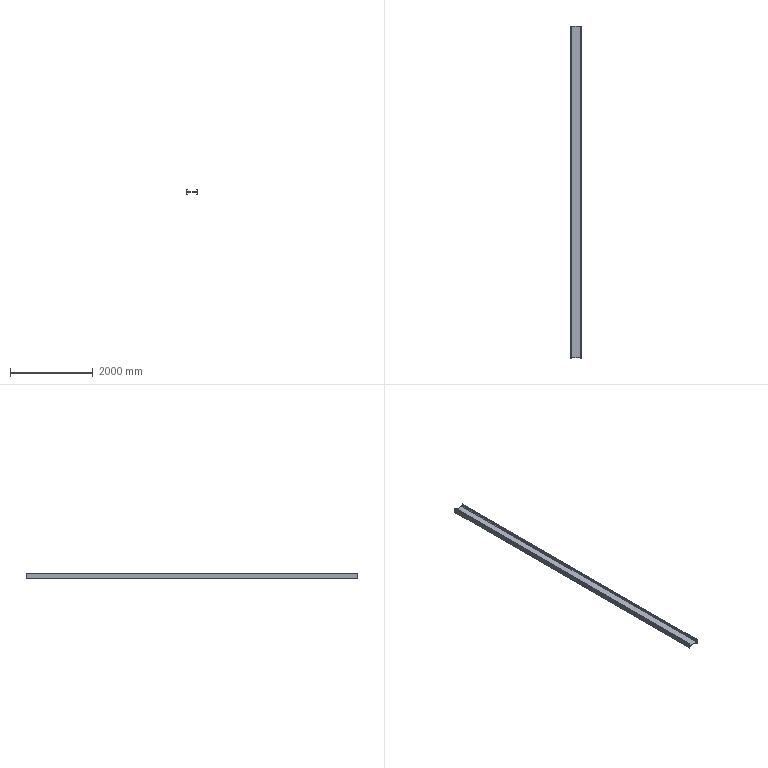Component | SolidWorks | H250X125-7375-16 | 1 solid | 18 faces | box 250 x 8000 x 125 mm | volume 30296567 mm3 | plane 14 | cylinder 4 | commonest cylinder face diameters 26 x4
build123d program:
from build123d import *

# Parameters (mm, degrees)
H_BEAM_HN250_125_1_DEPTH = 8000


with BuildPart() as part:
    # Sketch1 → H-Beam HN250_125_1 (new body)
    with BuildSketch(Plane.YZ):
        with BuildLine():
            Line((-62.5, -125), (-62.5, -116))
            Line((-62.5, -116), (-16, -116))
            ThreePointArc((-16, -116), (-6.808, -112.192), (-3, -103))
            Line((-3, -103), (-3, 103))
            ThreePointArc((-3, 103), (-6.808, 112.192), (-16, 116))
            Line((-16, 116), (-62.5, 116))
            Line((-62.5, 116), (-62.5, 125))
            Line((-62.5, 125), (62.5, 125))
            Line((62.5, 125), (62.5, 116))
            Line((62.5, 116), (16, 116))
            ThreePointArc((16, 116), (6.808, 112.192), (3, 103))
            Line((3, 103), (3, -103))
            ThreePointArc((3, -103), (6.808, -112.192), (16, -116))
            Line((16, -116), (62.5, -116))
            Line((62.5, -116), (62.5, -125))
            Line((62.5, -125), (-62.5, -125))
        make_face()
    extrude(amount=H_BEAM_HN250_125_1_DEPTH)


solid = part.part

# Placed as in the assembly
solid = solid.moved(Location((1944.926, 805.154, 161.5), (90, -90, 0)))
STEP:
#1=COLOUR_RGB('',0.7922,0.8196,0.9333);
#2=FILL_AREA_STYLE_COLOUR('',#1);
#3=FILL_AREA_STYLE('',(#2));
#4=SURFACE_STYLE_FILL_AREA(#3);
#5=SURFACE_SIDE_STYLE('',(#4));
#6=SURFACE_STYLE_USAGE(.BOTH.,#5);
#7=PRESENTATION_STYLE_ASSIGNMENT((#6));
#8=CARTESIAN_POINT('',(71.651,-283.262,3.898));
#9=VERTEX_POINT('',#8);
#10=CARTESIAN_POINT('',(71.651,-283.262,8.819));
#11=VERTEX_POINT('',#10);
#12=CARTESIAN_POINT('',(71.651,-283.262,8.819));
#13=DIRECTION('',(0.,0.,1.));
#14=VECTOR('',#13,39.37);
#15=LINE('',#12,#14);
#16=EDGE_CURVE('',#9,#11,#15,.T.);
#17=ORIENTED_EDGE('',*,*,#16,.T.);
#18=CARTESIAN_POINT('',(71.651,31.699,8.819));
#19=VERTEX_POINT('',#18);
#20=CARTESIAN_POINT('',(71.651,31.699,8.819));
#21=DIRECTION('',(-0.,-1.,0.));
#22=VECTOR('',#21,39.37);
#23=LINE('',#20,#22);
#24=EDGE_CURVE('',#19,#11,#23,.T.);
#25=ORIENTED_EDGE('',*,*,#24,.F.);
#26=CARTESIAN_POINT('',(71.651,31.699,3.898));
#27=VERTEX_POINT('',#26);
#28=CARTESIAN_POINT('',(71.651,31.699,8.819));
#29=DIRECTION('',(0.,0.,1.));
#30=VECTOR('',#29,39.37);
#31=LINE('',#28,#30);
#32=EDGE_CURVE('',#27,#19,#31,.T.);
#33=ORIENTED_EDGE('',*,*,#32,.F.);
#34=CARTESIAN_POINT('',(71.651,31.699,3.898));
#35=DIRECTION('',(-0.,-1.,0.));
#36=VECTOR('',#35,39.37);
#37=LINE('',#34,#36);
#38=EDGE_CURVE('',#27,#9,#37,.T.);
#39=ORIENTED_EDGE('',*,*,#38,.T.);
#40=EDGE_LOOP('',(#17,#25,#33,#39));
#41=FACE_OUTER_BOUND('',#40,.T.);
#42=CARTESIAN_POINT('',(71.651,31.699,8.819));
#43=DIRECTION('',(1.,-0.,-0.));
#44=DIRECTION('',(0.,1.,-0.));
#45=AXIS2_PLACEMENT_3D('',#42,#43,#44);
#46=PLANE('',#45);
#47=ADVANCED_FACE('',(#41),#46,.F.);
#48=CARTESIAN_POINT('',(72.005,-283.262,8.819));
#49=VERTEX_POINT('',#48);
#50=CARTESIAN_POINT('',(72.005,-283.262,8.819));
#51=DIRECTION('',(1.,-0.,-0.));
#52=VECTOR('',#51,39.37);
#53=LINE('',#50,#52);
#54=EDGE_CURVE('',#11,#49,#53,.T.);
#55=ORIENTED_EDGE('',*,*,#54,.T.);
#56=CARTESIAN_POINT('',(72.005,31.699,8.819));
#57=VERTEX_POINT('',#56);
#58=CARTESIAN_POINT('',(72.005,31.699,8.819));
#59=DIRECTION('',(-0.,-1.,0.));
#60=VECTOR('',#59,39.37);
#61=LINE('',#58,#60);
#62=EDGE_CURVE('',#57,#49,#61,.T.);
#63=ORIENTED_EDGE('',*,*,#62,.F.);
#64=CARTESIAN_POINT('',(72.005,31.699,8.819));
#65=DIRECTION('',(1.,-0.,-0.));
#66=VECTOR('',#65,39.37);
#67=LINE('',#64,#66);
#68=EDGE_CURVE('',#19,#57,#67,.T.);
#69=ORIENTED_EDGE('',*,*,#68,.F.);
#70=ORIENTED_EDGE('',*,*,#24,.T.);
#71=EDGE_LOOP('',(#55,#63,#69,#70));
#72=FACE_OUTER_BOUND('',#71,.T.);
#73=CARTESIAN_POINT('',(72.005,31.699,8.819));
#74=DIRECTION('',(-0.,-0.,-1.));
#75=DIRECTION('',(-1.,0.,0.));
#76=AXIS2_PLACEMENT_3D('',#73,#74,#75);
#77=PLANE('',#76);
#78=ADVANCED_FACE('',(#72),#77,.F.);
#79=CARTESIAN_POINT('',(72.005,-283.262,6.988));
#80=VERTEX_POINT('',#79);
#81=CARTESIAN_POINT('',(72.005,-283.262,8.819));
#82=DIRECTION('',(0.,-0.,-1.));
#83=VECTOR('',#82,39.37);
#84=LINE('',#81,#83);
#85=EDGE_CURVE('',#49,#80,#84,.T.);
#86=ORIENTED_EDGE('',*,*,#85,.T.);
#87=CARTESIAN_POINT('',(72.005,31.699,6.988));
#88=VERTEX_POINT('',#87);
#89=CARTESIAN_POINT('',(72.005,31.699,6.988));
#90=DIRECTION('',(-0.,-1.,0.));
#91=VECTOR('',#90,39.37);
#92=LINE('',#89,#91);
#93=EDGE_CURVE('',#88,#80,#92,.T.);
#94=ORIENTED_EDGE('',*,*,#93,.F.);
#95=CARTESIAN_POINT('',(72.005,31.699,8.819));
#96=DIRECTION('',(0.,-0.,-1.));
#97=VECTOR('',#96,39.37);
#98=LINE('',#95,#97);
#99=EDGE_CURVE('',#57,#88,#98,.T.);
#100=ORIENTED_EDGE('',*,*,#99,.F.);
#101=ORIENTED_EDGE('',*,*,#62,.T.);
#102=EDGE_LOOP('',(#86,#94,#100,#101));
#103=FACE_OUTER_BOUND('',#102,.T.);
#104=CARTESIAN_POINT('',(72.005,31.699,8.819));
#105=DIRECTION('',(-1.,0.,-0.));
#106=DIRECTION('',(-0.,0.,1.));
#107=AXIS2_PLACEMENT_3D('',#104,#105,#106);
#108=PLANE('',#107);
#109=ADVANCED_FACE('',(#103),#108,.F.);
#110=CARTESIAN_POINT('',(72.517,-283.262,6.476));
#111=VERTEX_POINT('',#110);
#112=CARTESIAN_POINT('',(72.517,-283.262,6.988));
#113=DIRECTION('',(-0.,-1.,0.));
#114=DIRECTION('',(1.,0.,0.));
#115=AXIS2_PLACEMENT_3D('',#112,#113,#114);
#116=CIRCLE('',#115,0.5118);
#117=EDGE_CURVE('',#80,#111,#116,.T.);
#118=ORIENTED_EDGE('',*,*,#117,.T.);
#119=CARTESIAN_POINT('',(72.517,31.699,6.476));
#120=VERTEX_POINT('',#119);
#121=CARTESIAN_POINT('',(72.517,31.699,6.476));
#122=DIRECTION('',(-0.,-1.,0.));
#123=VECTOR('',#122,39.37);
#124=LINE('',#121,#123);
#125=EDGE_CURVE('',#120,#111,#124,.T.);
#126=ORIENTED_EDGE('',*,*,#125,.F.);
#127=CARTESIAN_POINT('',(72.517,31.699,6.988));
#128=DIRECTION('',(-0.,-1.,0.));
#129=DIRECTION('',(1.,0.,0.));
#130=AXIS2_PLACEMENT_3D('',#127,#128,#129);
#131=CIRCLE('',#130,0.5118);
#132=EDGE_CURVE('',#88,#120,#131,.T.);
#133=ORIENTED_EDGE('',*,*,#132,.F.);
#134=ORIENTED_EDGE('',*,*,#93,.T.);
#135=EDGE_LOOP('',(#118,#126,#133,#134));
#136=FACE_OUTER_BOUND('',#135,.T.);
#137=CARTESIAN_POINT('',(72.517,31.699,6.988));
#138=DIRECTION('',(-0.,-1.,0.));
#139=DIRECTION('',(1.,0.,0.));
#140=AXIS2_PLACEMENT_3D('',#137,#138,#139);
#141=CYLINDRICAL_SURFACE('',#140,0.5118);
#142=ADVANCED_FACE('',(#136),#141,.F.);
#143=CARTESIAN_POINT('',(80.627,-283.262,6.476));
#144=VERTEX_POINT('',#143);
#145=CARTESIAN_POINT('',(80.627,-283.262,6.476));
#146=DIRECTION('',(1.,-0.,-0.));
#147=VECTOR('',#146,39.37);
#148=LINE('',#145,#147);
#149=EDGE_CURVE('',#111,#144,#148,.T.);
#150=ORIENTED_EDGE('',*,*,#149,.T.);
#151=CARTESIAN_POINT('',(80.627,31.699,6.476));
#152=VERTEX_POINT('',#151);
#153=CARTESIAN_POINT('',(80.627,31.699,6.476));
#154=DIRECTION('',(-0.,-1.,0.));
#155=VECTOR('',#154,39.37);
#156=LINE('',#153,#155);
#157=EDGE_CURVE('',#152,#144,#156,.T.);
#158=ORIENTED_EDGE('',*,*,#157,.F.);
#159=CARTESIAN_POINT('',(80.627,31.699,6.476));
#160=DIRECTION('',(1.,-0.,-0.));
#161=VECTOR('',#160,39.37);
#162=LINE('',#159,#161);
#163=EDGE_CURVE('',#120,#152,#162,.T.);
#164=ORIENTED_EDGE('',*,*,#163,.F.);
#165=ORIENTED_EDGE('',*,*,#125,.T.);
#166=EDGE_LOOP('',(#150,#158,#164,#165));
#167=FACE_OUTER_BOUND('',#166,.T.);
#168=CARTESIAN_POINT('',(80.627,31.699,6.476));
#169=DIRECTION('',(-0.,-0.,-1.));
#170=DIRECTION('',(-1.,0.,0.));
#171=AXIS2_PLACEMENT_3D('',#168,#169,#170);
#172=PLANE('',#171);
#173=ADVANCED_FACE('',(#167),#172,.F.);
#174=CARTESIAN_POINT('',(81.139,-283.262,6.988));
#175=VERTEX_POINT('',#174);
#176=CARTESIAN_POINT('',(80.627,-283.262,6.988));
#177=DIRECTION('',(-0.,-1.,0.));
#178=DIRECTION('',(1.,0.,0.));
#179=AXIS2_PLACEMENT_3D('',#176,#177,#178);
#180=CIRCLE('',#179,0.5118);
#181=EDGE_CURVE('',#144,#175,#180,.T.);
#182=ORIENTED_EDGE('',*,*,#181,.T.);
#183=CARTESIAN_POINT('',(81.139,31.699,6.988));
#184=VERTEX_POINT('',#183);
#185=CARTESIAN_POINT('',(81.139,31.699,6.988));
#186=DIRECTION('',(-0.,-1.,0.));
#187=VECTOR('',#186,39.37);
#188=LINE('',#185,#187);
#189=EDGE_CURVE('',#184,#175,#188,.T.);
#190=ORIENTED_EDGE('',*,*,#189,.F.);
#191=CARTESIAN_POINT('',(80.627,31.699,6.988));
#192=DIRECTION('',(-0.,-1.,0.));
#193=DIRECTION('',(1.,0.,0.));
#194=AXIS2_PLACEMENT_3D('',#191,#192,#193);
#195=CIRCLE('',#194,0.5118);
#196=EDGE_CURVE('',#152,#184,#195,.T.);
#197=ORIENTED_EDGE('',*,*,#196,.F.);
#198=ORIENTED_EDGE('',*,*,#157,.T.);
#199=EDGE_LOOP('',(#182,#190,#197,#198));
#200=FACE_OUTER_BOUND('',#199,.T.);
#201=CARTESIAN_POINT('',(80.627,31.699,6.988));
#202=DIRECTION('',(-0.,-1.,0.));
#203=DIRECTION('',(1.,0.,0.));
#204=AXIS2_PLACEMENT_3D('',#201,#202,#203);
#205=CYLINDRICAL_SURFACE('',#204,0.5118);
#206=ADVANCED_FACE('',(#200),#205,.F.);
#207=CARTESIAN_POINT('',(81.139,-283.262,8.819));
#208=VERTEX_POINT('',#207);
#209=CARTESIAN_POINT('',(81.139,-283.262,6.988));
#210=DIRECTION('',(0.,0.,1.));
#211=VECTOR('',#210,39.37);
#212=LINE('',#209,#211);
#213=EDGE_CURVE('',#175,#208,#212,.T.);
#214=ORIENTED_EDGE('',*,*,#213,.T.);
#215=CARTESIAN_POINT('',(81.139,31.699,8.819));
#216=VERTEX_POINT('',#215);
#217=CARTESIAN_POINT('',(81.139,31.699,8.819));
#218=DIRECTION('',(-0.,-1.,0.));
#219=VECTOR('',#218,39.37);
#220=LINE('',#217,#219);
#221=EDGE_CURVE('',#216,#208,#220,.T.);
#222=ORIENTED_EDGE('',*,*,#221,.F.);
#223=CARTESIAN_POINT('',(81.139,31.699,6.988));
#224=DIRECTION('',(0.,0.,1.));
#225=VECTOR('',#224,39.37);
#226=LINE('',#223,#225);
#227=EDGE_CURVE('',#184,#216,#226,.T.);
#228=ORIENTED_EDGE('',*,*,#227,.F.);
#229=ORIENTED_EDGE('',*,*,#189,.T.);
#230=EDGE_LOOP('',(#214,#222,#228,#229));
#231=FACE_OUTER_BOUND('',#230,.T.);
#232=CARTESIAN_POINT('',(81.139,31.699,6.988));
#233=DIRECTION('',(1.,-0.,-0.));
#234=DIRECTION('',(0.,1.,-0.));
#235=AXIS2_PLACEMENT_3D('',#232,#233,#234);
#236=PLANE('',#235);
#237=ADVANCED_FACE('',(#231),#236,.F.);
#238=CARTESIAN_POINT('',(81.493,-283.262,8.819));
#239=VERTEX_POINT('',#238);
#240=CARTESIAN_POINT('',(81.493,-283.262,8.819));
#241=DIRECTION('',(1.,-0.,-0.));
#242=VECTOR('',#241,39.37);
#243=LINE('',#240,#242);
#244=EDGE_CURVE('',#208,#239,#243,.T.);
#245=ORIENTED_EDGE('',*,*,#244,.T.);
#246=CARTESIAN_POINT('',(81.493,31.699,8.819));
#247=VERTEX_POINT('',#246);
#248=CARTESIAN_POINT('',(81.493,31.699,8.819));
#249=DIRECTION('',(-0.,-1.,0.));
#250=VECTOR('',#249,39.37);
#251=LINE('',#248,#250);
#252=EDGE_CURVE('',#247,#239,#251,.T.);
#253=ORIENTED_EDGE('',*,*,#252,.F.);
#254=CARTESIAN_POINT('',(81.493,31.699,8.819));
#255=DIRECTION('',(1.,-0.,-0.));
#256=VECTOR('',#255,39.37);
#257=LINE('',#254,#256);
#258=EDGE_CURVE('',#216,#247,#257,.T.);
#259=ORIENTED_EDGE('',*,*,#258,.F.);
#260=ORIENTED_EDGE('',*,*,#221,.T.);
#261=EDGE_LOOP('',(#245,#253,#259,#260));
#262=FACE_OUTER_BOUND('',#261,.T.);
#263=CARTESIAN_POINT('',(81.493,31.699,8.819));
#264=DIRECTION('',(-0.,-0.,-1.));
#265=DIRECTION('',(-1.,0.,0.));
#266=AXIS2_PLACEMENT_3D('',#263,#264,#265);
#267=PLANE('',#266);
#268=ADVANCED_FACE('',(#262),#267,.F.);
#269=CARTESIAN_POINT('',(81.493,-283.262,3.898));
#270=VERTEX_POINT('',#269);
#271=CARTESIAN_POINT('',(81.493,-283.262,3.898));
#272=DIRECTION('',(-0.,-0.,-1.));
#273=VECTOR('',#272,39.37);
#274=LINE('',#271,#273);
#275=EDGE_CURVE('',#239,#270,#274,.T.);
#276=ORIENTED_EDGE('',*,*,#275,.T.);
#277=CARTESIAN_POINT('',(81.493,31.699,3.898));
#278=VERTEX_POINT('',#277);
#279=CARTESIAN_POINT('',(81.493,31.699,3.898));
#280=DIRECTION('',(-0.,-1.,0.));
#281=VECTOR('',#280,39.37);
#282=LINE('',#279,#281);
#283=EDGE_CURVE('',#278,#270,#282,.T.);
#284=ORIENTED_EDGE('',*,*,#283,.F.);
#285=CARTESIAN_POINT('',(81.493,31.699,3.898));
#286=DIRECTION('',(-0.,-0.,-1.));
#287=VECTOR('',#286,39.37);
#288=LINE('',#285,#287);
#289=EDGE_CURVE('',#247,#278,#288,.T.);
#290=ORIENTED_EDGE('',*,*,#289,.F.);
#291=ORIENTED_EDGE('',*,*,#252,.T.);
#292=EDGE_LOOP('',(#276,#284,#290,#291));
#293=FACE_OUTER_BOUND('',#292,.T.);
#294=CARTESIAN_POINT('',(81.493,31.699,3.898));
#295=DIRECTION('',(-1.,0.,0.));
#296=DIRECTION('',(-0.,-1.,0.));
#297=AXIS2_PLACEMENT_3D('',#294,#295,#296);
#298=PLANE('',#297);
#299=ADVANCED_FACE('',(#293),#298,.F.);
#300=CARTESIAN_POINT('',(81.139,-283.262,3.898));
#301=VERTEX_POINT('',#300);
#302=CARTESIAN_POINT('',(81.139,-283.262,3.898));
#303=DIRECTION('',(-1.,0.,0.));
#304=VECTOR('',#303,39.37);
#305=LINE('',#302,#304);
#306=EDGE_CURVE('',#270,#301,#305,.T.);
#307=ORIENTED_EDGE('',*,*,#306,.T.);
#308=CARTESIAN_POINT('',(81.139,31.699,3.898));
#309=VERTEX_POINT('',#308);
#310=CARTESIAN_POINT('',(81.139,31.699,3.898));
#311=DIRECTION('',(-0.,-1.,0.));
#312=VECTOR('',#311,39.37);
#313=LINE('',#310,#312);
#314=EDGE_CURVE('',#309,#301,#313,.T.);
#315=ORIENTED_EDGE('',*,*,#314,.F.);
#316=CARTESIAN_POINT('',(81.139,31.699,3.898));
#317=DIRECTION('',(-1.,0.,0.));
#318=VECTOR('',#317,39.37);
#319=LINE('',#316,#318);
#320=EDGE_CURVE('',#278,#309,#319,.T.);
#321=ORIENTED_EDGE('',*,*,#320,.F.);
#322=ORIENTED_EDGE('',*,*,#283,.T.);
#323=EDGE_LOOP('',(#307,#315,#321,#322));
#324=FACE_OUTER_BOUND('',#323,.T.);
#325=CARTESIAN_POINT('',(81.139,31.699,3.898));
#326=DIRECTION('',(0.,0.,1.));
#327=DIRECTION('',(1.,-0.,-0.));
#328=AXIS2_PLACEMENT_3D('',#325,#326,#327);
#329=PLANE('',#328);
#330=ADVANCED_FACE('',(#324),#329,.F.);
#331=CARTESIAN_POINT('',(81.139,-283.262,5.728));
#332=VERTEX_POINT('',#331);
#333=CARTESIAN_POINT('',(81.139,-283.262,3.898));
#334=DIRECTION('',(0.,0.,1.));
#335=VECTOR('',#334,39.37);
#336=LINE('',#333,#335);
#337=EDGE_CURVE('',#301,#332,#336,.T.);
#338=ORIENTED_EDGE('',*,*,#337,.T.);
#339=CARTESIAN_POINT('',(81.139,31.699,5.728));
#340=VERTEX_POINT('',#339);
#341=CARTESIAN_POINT('',(81.139,31.699,5.728));
#342=DIRECTION('',(-0.,-1.,0.));
#343=VECTOR('',#342,39.37);
#344=LINE('',#341,#343);
#345=EDGE_CURVE('',#340,#332,#344,.T.);
#346=ORIENTED_EDGE('',*,*,#345,.F.);
#347=CARTESIAN_POINT('',(81.139,31.699,3.898));
#348=DIRECTION('',(0.,0.,1.));
#349=VECTOR('',#348,39.37);
#350=LINE('',#347,#349);
#351=EDGE_CURVE('',#309,#340,#350,.T.);
#352=ORIENTED_EDGE('',*,*,#351,.F.);
#353=ORIENTED_EDGE('',*,*,#314,.T.);
#354=EDGE_LOOP('',(#338,#346,#352,#353));
#355=FACE_OUTER_BOUND('',#354,.T.);
#356=CARTESIAN_POINT('',(81.139,31.699,3.898));
#357=DIRECTION('',(1.,-0.,-0.));
#358=DIRECTION('',(0.,1.,-0.));
#359=AXIS2_PLACEMENT_3D('',#356,#357,#358);
#360=PLANE('',#359);
#361=ADVANCED_FACE('',(#355),#360,.F.);
#362=CARTESIAN_POINT('',(80.627,-283.262,6.24));
#363=VERTEX_POINT('',#362);
#364=CARTESIAN_POINT('',(80.627,-283.262,5.728));
#365=DIRECTION('',(-0.,-1.,0.));
#366=DIRECTION('',(-1.,0.,0.));
#367=AXIS2_PLACEMENT_3D('',#364,#365,#366);
#368=CIRCLE('',#367,0.5118);
#369=EDGE_CURVE('',#332,#363,#368,.T.);
#370=ORIENTED_EDGE('',*,*,#369,.T.);
#371=CARTESIAN_POINT('',(80.627,31.699,6.24));
#372=VERTEX_POINT('',#371);
#373=CARTESIAN_POINT('',(80.627,31.699,6.24));
#374=DIRECTION('',(-0.,-1.,0.));
#375=VECTOR('',#374,39.37);
#376=LINE('',#373,#375);
#377=EDGE_CURVE('',#372,#363,#376,.T.);
#378=ORIENTED_EDGE('',*,*,#377,.F.);
#379=CARTESIAN_POINT('',(80.627,31.699,5.728));
#380=DIRECTION('',(-0.,-1.,0.));
#381=DIRECTION('',(-1.,0.,0.));
#382=AXIS2_PLACEMENT_3D('',#379,#380,#381);
#383=CIRCLE('',#382,0.5118);
#384=EDGE_CURVE('',#340,#372,#383,.T.);
#385=ORIENTED_EDGE('',*,*,#384,.F.);
#386=ORIENTED_EDGE('',*,*,#345,.T.);
#387=EDGE_LOOP('',(#370,#378,#385,#386));
#388=FACE_OUTER_BOUND('',#387,.T.);
#389=CARTESIAN_POINT('',(80.627,31.699,5.728));
#390=DIRECTION('',(-0.,-1.,0.));
#391=DIRECTION('',(1.,0.,0.));
#392=AXIS2_PLACEMENT_3D('',#389,#390,#391);
#393=CYLINDRICAL_SURFACE('',#392,0.5118);
#394=ADVANCED_FACE('',(#388),#393,.F.);
#395=CARTESIAN_POINT('',(72.517,-283.262,6.24));
#396=VERTEX_POINT('',#395);
#397=CARTESIAN_POINT('',(72.517,-283.262,6.24));
#398=DIRECTION('',(-1.,0.,0.));
#399=VECTOR('',#398,39.37);
#400=LINE('',#397,#399);
#401=EDGE_CURVE('',#363,#396,#400,.T.);
#402=ORIENTED_EDGE('',*,*,#401,.T.);
#403=CARTESIAN_POINT('',(72.517,31.699,6.24));
#404=VERTEX_POINT('',#403);
#405=CARTESIAN_POINT('',(72.517,31.699,6.24));
#406=DIRECTION('',(-0.,-1.,0.));
#407=VECTOR('',#406,39.37);
#408=LINE('',#405,#407);
#409=EDGE_CURVE('',#404,#396,#408,.T.);
#410=ORIENTED_EDGE('',*,*,#409,.F.);
#411=CARTESIAN_POINT('',(72.517,31.699,6.24));
#412=DIRECTION('',(-1.,0.,0.));
#413=VECTOR('',#412,39.37);
#414=LINE('',#411,#413);
#415=EDGE_CURVE('',#372,#404,#414,.T.);
#416=ORIENTED_EDGE('',*,*,#415,.F.);
#417=ORIENTED_EDGE('',*,*,#377,.T.);
#418=EDGE_LOOP('',(#402,#410,#416,#417));
#419=FACE_OUTER_BOUND('',#418,.T.);
#420=CARTESIAN_POINT('',(72.517,31.699,6.24));
#421=DIRECTION('',(0.,0.,1.));
#422=DIRECTION('',(1.,-0.,-0.));
#423=AXIS2_PLACEMENT_3D('',#420,#421,#422);
#424=PLANE('',#423);
#425=ADVANCED_FACE('',(#419),#424,.F.);
#426=CARTESIAN_POINT('',(72.005,-283.262,5.728));
#427=VERTEX_POINT('',#426);
#428=CARTESIAN_POINT('',(72.517,-283.262,5.728));
#429=DIRECTION('',(-0.,-1.,0.));
#430=DIRECTION('',(-1.,0.,0.));
#431=AXIS2_PLACEMENT_3D('',#428,#429,#430);
#432=CIRCLE('',#431,0.5118);
#433=EDGE_CURVE('',#396,#427,#432,.T.);
#434=ORIENTED_EDGE('',*,*,#433,.T.);
#435=CARTESIAN_POINT('',(72.005,31.699,5.728));
#436=VERTEX_POINT('',#435);
#437=CARTESIAN_POINT('',(72.005,31.699,5.728));
#438=DIRECTION('',(-0.,-1.,0.));
#439=VECTOR('',#438,39.37);
#440=LINE('',#437,#439);
#441=EDGE_CURVE('',#436,#427,#440,.T.);
#442=ORIENTED_EDGE('',*,*,#441,.F.);
#443=CARTESIAN_POINT('',(72.517,31.699,5.728));
#444=DIRECTION('',(-0.,-1.,0.));
#445=DIRECTION('',(-1.,0.,0.));
#446=AXIS2_PLACEMENT_3D('',#443,#444,#445);
#447=CIRCLE('',#446,0.5118);
#448=EDGE_CURVE('',#404,#436,#447,.T.);
#449=ORIENTED_EDGE('',*,*,#448,.F.);
#450=ORIENTED_EDGE('',*,*,#409,.T.);
#451=EDGE_LOOP('',(#434,#442,#449,#450));
#452=FACE_OUTER_BOUND('',#451,.T.);
#453=CARTESIAN_POINT('',(72.517,31.699,5.728));
#454=DIRECTION('',(-0.,-1.,0.));
#455=DIRECTION('',(1.,0.,0.));
#456=AXIS2_PLACEMENT_3D('',#453,#454,#455);
#457=CYLINDRICAL_SURFACE('',#456,0.5118);
#458=ADVANCED_FACE('',(#452),#457,.F.);
#459=CARTESIAN_POINT('',(72.005,-283.262,3.898));
#460=VERTEX_POINT('',#459);
#461=CARTESIAN_POINT('',(72.005,-283.262,5.728));
#462=DIRECTION('',(-0.,-0.,-1.));
#463=VECTOR('',#462,39.37);
#464=LINE('',#461,#463);
#465=EDGE_CURVE('',#427,#460,#464,.T.);
#466=ORIENTED_EDGE('',*,*,#465,.T.);
#467=CARTESIAN_POINT('',(72.005,31.699,3.898));
#468=VERTEX_POINT('',#467);
#469=CARTESIAN_POINT('',(72.005,31.699,3.898));
#470=DIRECTION('',(-0.,-1.,0.));
#471=VECTOR('',#470,39.37);
#472=LINE('',#469,#471);
#473=EDGE_CURVE('',#468,#460,#472,.T.);
#474=ORIENTED_EDGE('',*,*,#473,.F.);
#475=CARTESIAN_POINT('',(72.005,31.699,5.728));
#476=DIRECTION('',(-0.,-0.,-1.));
#477=VECTOR('',#476,39.37);
#478=LINE('',#475,#477);
#479=EDGE_CURVE('',#436,#468,#478,.T.);
#480=ORIENTED_EDGE('',*,*,#479,.F.);
#481=ORIENTED_EDGE('',*,*,#441,.T.);
#482=EDGE_LOOP('',(#466,#474,#480,#481));
#483=FACE_OUTER_BOUND('',#482,.T.);
#484=CARTESIAN_POINT('',(72.005,31.699,5.728));
#485=DIRECTION('',(-1.,0.,0.));
#486=DIRECTION('',(0.,0.,1.));
#487=AXIS2_PLACEMENT_3D('',#484,#485,#486);
#488=PLANE('',#487);
#489=ADVANCED_FACE('',(#483),#488,.F.);
#490=CARTESIAN_POINT('',(71.651,-283.262,3.898));
#491=DIRECTION('',(-1.,0.,0.));
#492=VECTOR('',#491,39.37);
#493=LINE('',#490,#492);
#494=EDGE_CURVE('',#460,#9,#493,.T.);
#495=ORIENTED_EDGE('',*,*,#494,.T.);
#496=ORIENTED_EDGE('',*,*,#38,.F.);
#497=CARTESIAN_POINT('',(71.651,31.699,3.898));
#498=DIRECTION('',(-1.,0.,0.));
#499=VECTOR('',#498,39.37);
#500=LINE('',#497,#499);
#501=EDGE_CURVE('',#468,#27,#500,.T.);
#502=ORIENTED_EDGE('',*,*,#501,.F.);
#503=ORIENTED_EDGE('',*,*,#473,.T.);
#504=EDGE_LOOP('',(#495,#496,#502,#503));
#505=FACE_OUTER_BOUND('',#504,.T.);
#506=CARTESIAN_POINT('',(71.651,31.699,3.898));
#507=DIRECTION('',(0.,0.,1.));
#508=DIRECTION('',(1.,-0.,-0.));
#509=AXIS2_PLACEMENT_3D('',#506,#507,#508);
#510=PLANE('',#509);
#511=ADVANCED_FACE('',(#505),#510,.F.);
#512=ORIENTED_EDGE('',*,*,#32,.T.);
#513=ORIENTED_EDGE('',*,*,#68,.T.);
#514=ORIENTED_EDGE('',*,*,#99,.T.);
#515=ORIENTED_EDGE('',*,*,#132,.T.);
#516=ORIENTED_EDGE('',*,*,#163,.T.);
#517=ORIENTED_EDGE('',*,*,#196,.T.);
#518=ORIENTED_EDGE('',*,*,#227,.T.);
#519=ORIENTED_EDGE('',*,*,#258,.T.);
#520=ORIENTED_EDGE('',*,*,#289,.T.);
#521=ORIENTED_EDGE('',*,*,#320,.T.);
#522=ORIENTED_EDGE('',*,*,#351,.T.);
#523=ORIENTED_EDGE('',*,*,#384,.T.);
#524=ORIENTED_EDGE('',*,*,#415,.T.);
#525=ORIENTED_EDGE('',*,*,#448,.T.);
#526=ORIENTED_EDGE('',*,*,#479,.T.);
#527=ORIENTED_EDGE('',*,*,#501,.T.);
#528=EDGE_LOOP('',(#512,#513,#514,#515,#516,#517,#518,#519,#520,#521,#522,#523,#524,#525,#526,#527));
#529=FACE_OUTER_BOUND('',#528,.T.);
#530=CARTESIAN_POINT('',(72.517,31.699,5.728));
#531=DIRECTION('',(0.,1.,-0.));
#532=DIRECTION('',(-1.,0.,0.));
#533=AXIS2_PLACEMENT_3D('',#530,#531,#532);
#534=PLANE('',#533);
#535=ADVANCED_FACE('',(#529),#534,.T.);
#536=ORIENTED_EDGE('',*,*,#16,.F.);
#537=ORIENTED_EDGE('',*,*,#494,.F.);
#538=ORIENTED_EDGE('',*,*,#465,.F.);
#539=ORIENTED_EDGE('',*,*,#433,.F.);
#540=ORIENTED_EDGE('',*,*,#401,.F.);
#541=ORIENTED_EDGE('',*,*,#369,.F.);
#542=ORIENTED_EDGE('',*,*,#337,.F.);
#543=ORIENTED_EDGE('',*,*,#306,.F.);
#544=ORIENTED_EDGE('',*,*,#275,.F.);
#545=ORIENTED_EDGE('',*,*,#244,.F.);
#546=ORIENTED_EDGE('',*,*,#213,.F.);
#547=ORIENTED_EDGE('',*,*,#181,.F.);
#548=ORIENTED_EDGE('',*,*,#149,.F.);
#549=ORIENTED_EDGE('',*,*,#117,.F.);
#550=ORIENTED_EDGE('',*,*,#85,.F.);
#551=ORIENTED_EDGE('',*,*,#54,.F.);
#552=EDGE_LOOP('',(#536,#537,#538,#539,#540,#541,#542,#543,#544,#545,#546,#547,#548,#549,#550,#551));
#553=FACE_OUTER_BOUND('',#552,.T.);
#554=CARTESIAN_POINT('',(72.517,-283.262,5.728));
#555=DIRECTION('',(0.,1.,-0.));
#556=DIRECTION('',(-1.,0.,0.));
#557=AXIS2_PLACEMENT_3D('',#554,#555,#556);
#558=PLANE('',#557);
#559=ADVANCED_FACE('',(#553),#558,.F.);
#560=CLOSED_SHELL('',(#47,#78,#109,#142,#173,#206,#237,#268,#299,#330,#361,#394,#425,#458,#489,#511,#535,#559));
#561=MANIFOLD_SOLID_BREP('',#560);
#562=STYLED_ITEM('',(#7),#561);
#563=(LENGTH_UNIT()NAMED_UNIT(*)SI_UNIT($,.METRE.));
#564=LENGTH_MEASURE_WITH_UNIT(LENGTH_MEASURE(0.0254),#563);
#565=DIMENSIONAL_EXPONENTS(1.,0.,0.,0.,0.,0.,0.);
#566=(CONVERSION_BASED_UNIT('',#564)LENGTH_UNIT()NAMED_UNIT(#565));
#567=UNCERTAINTY_MEASURE_WITH_UNIT(LENGTH_MEASURE(0.00001),#566,'','');
#568=(NAMED_UNIT(*)PLANE_ANGLE_UNIT()SI_UNIT($,.RADIAN.));
#569=(NAMED_UNIT(*)SI_UNIT($,.STERADIAN.)SOLID_ANGLE_UNIT());
#570=(GEOMETRIC_REPRESENTATION_CONTEXT(3)GLOBAL_UNCERTAINTY_ASSIGNED_CONTEXT((#567))GLOBAL_UNIT_ASSIGNED_CONTEXT((#566,#568,#569))REPRESENTATION_CONTEXT('',''));
#571=MECHANICAL_DESIGN_GEOMETRIC_PRESENTATION_REPRESENTATION('',(#562),#570);
#572=PRESENTATION_LAYER_ASSIGNMENT('','',(#562));
#573=CARTESIAN_POINT('',(0.,0.,0.));
#574=DIRECTION('',(0.,0.,1.));
#575=DIRECTION('',(1.,0.,0.));
#576=AXIS2_PLACEMENT_3D('',#573,#574,#575);
#577=(LENGTH_UNIT()NAMED_UNIT(*)SI_UNIT($,.METRE.));
#578=LENGTH_MEASURE_WITH_UNIT(LENGTH_MEASURE(0.0254),#577);
#579=DIMENSIONAL_EXPONENTS(1.,0.,0.,0.,0.,0.,0.);
#580=(CONVERSION_BASED_UNIT('',#578)LENGTH_UNIT()NAMED_UNIT(#579));
#581=UNCERTAINTY_MEASURE_WITH_UNIT(LENGTH_MEASURE(0.00001),#580,'','');
#582=(NAMED_UNIT(*)PLANE_ANGLE_UNIT()SI_UNIT($,.RADIAN.));
#583=(NAMED_UNIT(*)SI_UNIT($,.STERADIAN.)SOLID_ANGLE_UNIT());
#584=(GEOMETRIC_REPRESENTATION_CONTEXT(3)GLOBAL_UNCERTAINTY_ASSIGNED_CONTEXT((#581))GLOBAL_UNIT_ASSIGNED_CONTEXT((#580,#582,#583))REPRESENTATION_CONTEXT('',''));
#585=ADVANCED_BREP_SHAPE_REPRESENTATION('',(#561,#576),#584);